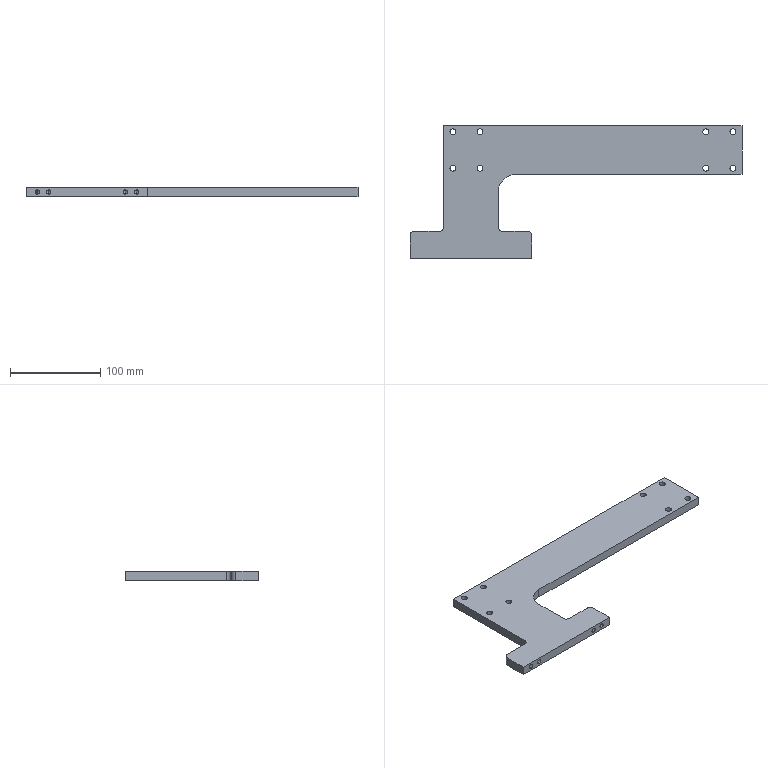Component | SolidWorks | CTM-HVS-42-02-29-1 | 1 solid | 57 faces | box 367.5 x 147 x 10 mm | volume 252599 mm3 | cylinder 33 | cone 12 | plane 12 | commonest cylinder face diameters 6.6 x16 5 x12 10 x4 40 x1 | material Q235A
build123d program:
from build123d import *

# Parameters (mm, degrees)
EXTRUDE1_DEPTH        = 5
FILLET1_R             = 20
SKETCH2_R             = 3.3
EXTRUDE2_DEPTH        = 362.399
LPATTERN1_COUNT       = 2
LPATTERN1_PITCH       = 250
LPATTERN2_COUNT       = 2
LPATTERN2_PITCH       = 40
LPATTERN3_COUNT       = 2
LPATTERN3_PITCH       = 310
LPATTERN4_COUNT       = 2
LPATTERN4_PITCH       = 35
FILLET2_R             = 5
M6_TAPPED_HOLE3_D     = 5
M6_TAPPED_HOLE3_DEPTH = 15
M6_TAPPED_HOLE3_TIP   = 1.502
FILLET3_R             = 5


with BuildPart() as part:
    # Sketch1 → Extrude1 (new, symmetric)
    with BuildSketch(Plane.XY):
        Polygon((0, 30), (0, 147), (330, 147), (330, 93), (60, 93), (60, 30), (97.5, 30), (97.5, 0), (60, 0), (0, 0), (-37.5, 0), (-37.5, 30), align=None)
    extrude(amount=EXTRUDE1_DEPTH, both=True)

    # Fillet1
    fillet1_edges = [part.edges().sort_by_distance(p)[0] for p in [
        (60, 93, 0),
    ]]
    fillet(fillet1_edges, radius=FILLET1_R)

    # Sketch2 → Extrude2 (cut, through all)
    with BuildSketch(Plane.XY.offset(5)):
        with Locations((40, 140)):
            Circle(SKETCH2_R)
        with Locations((40, 100)):
            Circle(SKETCH2_R)
    extrude2 = extrude(amount=-EXTRUDE2_DEPTH, mode=Mode.SUBTRACT)

    # LPattern1: Extrude2 ×2
    with Locations(*[(i * LPATTERN1_PITCH, 0, 0) for i in range(1, LPATTERN1_COUNT)]):
        add(extrude2, mode=Mode.SUBTRACT)

    # Sketch5 → M6 Clearance Hole1 (revolve, cut)
    with BuildSketch(Plane(origin=(10, 140, 5), x_dir=(0, -1, 0), z_dir=(1, 0, 0))):
        Polygon((0, 0), (0, 36.983), (3.3, 35), (3.3, 0), align=None)
    m6_clearance_hole1 = revolve(axis=Axis((10, 140, 11.35), (0, 0, -1)), mode=Mode.SUBTRACT)

    # LPattern2: M6 Clearance Hole1 ×2
    with Locations(*[(0, -i * LPATTERN2_PITCH, 0) for i in range(1, LPATTERN2_COUNT)]):
        add(m6_clearance_hole1, mode=Mode.SUBTRACT)

    # LPattern3: M6 Clearance Hole1 ×2
    with Locations(*[(i * LPATTERN3_PITCH, 0, 0) for i in range(1, LPATTERN3_COUNT)]):
        add(m6_clearance_hole1, mode=Mode.SUBTRACT)

    # LPattern3 copy 1 sketch → LPattern3 copy 1 (revolve, cut)
    with BuildSketch(Plane(origin=(320, 100, 5), x_dir=(0, -1, 0), z_dir=(1, 0, 0))):
        Polygon((0, 0), (0, 36.983), (3.3, 35), (3.3, 0), align=None)
    revolve(axis=Axis((320, 100, 11.35), (0, 0, -1)), mode=Mode.SUBTRACT)

    # Sketch6 → M6 Tapped Hole2 (revolve, cut)
    with BuildSketch(Plane(origin=(17.5, 147, 0), x_dir=(0, 0, 1), z_dir=(1, 0, 0))):
        Polygon((0, 0), (0, 21.502), (2.5, 20), (2.5, 0), align=None)
    m6_tapped_hole2 = revolve(axis=Axis((17.5, 153.35, 0), (0, -1, 0)), mode=Mode.SUBTRACT)

    # LPattern4: M6 Tapped Hole2 ×2
    with Locations(*[(i * LPATTERN4_PITCH, 0, 0) for i in range(1, LPATTERN4_COUNT)]):
        add(m6_tapped_hole2, mode=Mode.SUBTRACT)

    # Fillet2
    fillet2_edges = [part.edges().sort_by_distance(p)[0] for p in [
        (0, 30, 0),
        (60, 30, 0),
    ]]
    fillet(fillet2_edges, radius=FILLET2_R)

    # M6 Tapped Hole3
    with Locations(Plane.XZ):
        with Locations((-12.5, 0), (72.5, 0), (85, 0), (-25, 0)):
            Hole(M6_TAPPED_HOLE3_D / 2, depth=M6_TAPPED_HOLE3_DEPTH)
            with Locations((0, 0, -(M6_TAPPED_HOLE3_DEPTH + M6_TAPPED_HOLE3_TIP / 2))):  # 118° drill point
                Cone(0, M6_TAPPED_HOLE3_D / 2, M6_TAPPED_HOLE3_TIP, mode=Mode.SUBTRACT)

    # Fillet3
    fillet3_edges = [part.edges().sort_by_distance(p)[0] for p in [
        (-37.5, 30, 0),
        (97.5, 30, 0),
    ]]
    fillet(fillet3_edges, radius=FILLET3_R)


solid = part.part

# Placed as in the assembly
solid = solid.moved(Location((-322.307, -64.557, 0), (0, 0, 0)))